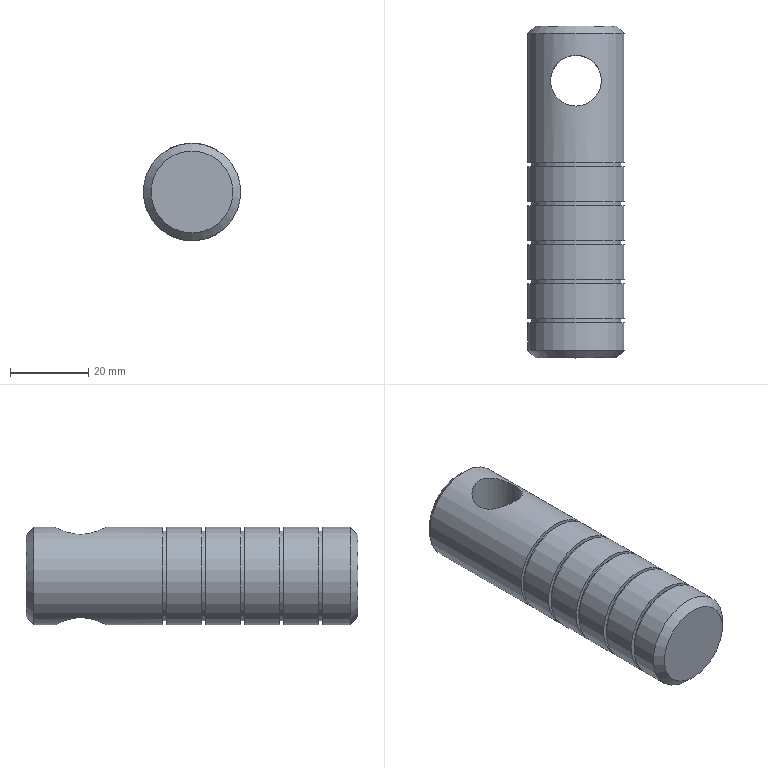Component | NX | 11_PLUNGER | 1 solid | 26 faces | volume 37849 mm3 | plane 12 | cylinder 12 | cone 2 | commonest cylinder face diameters 25 x6 23 x5 13 x1